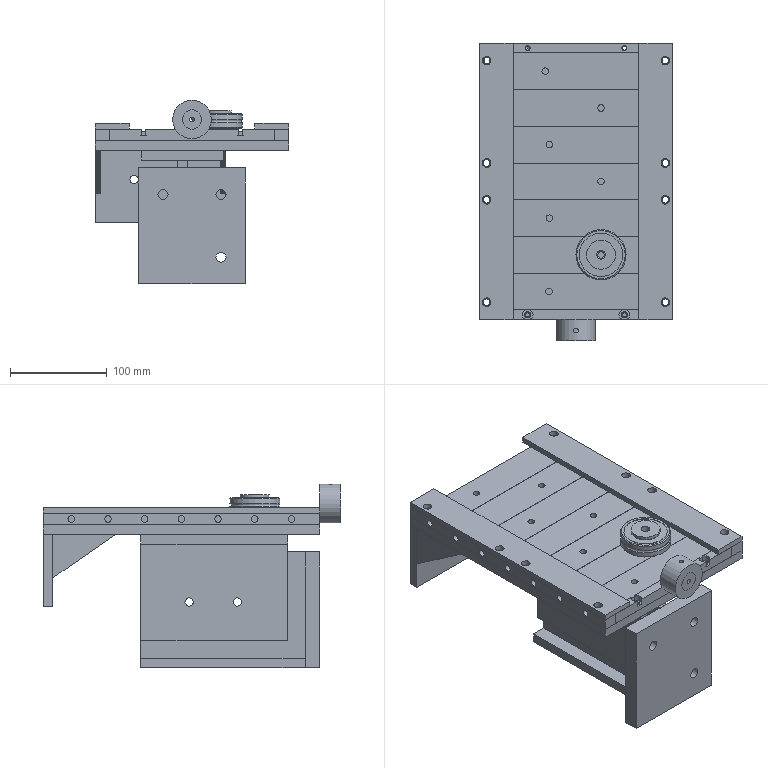Assembly | NX | mm | 25 component files | 25 solids | 279 faces | box 200 x 308 x 190.07 mm | volume 2075251 mm3 | plane 144 | cylinder 95 | cone 39 | torus 1 | commonest cylinder face diameters 6.8 x36 9 x17 10.5 x11 20 x5 4.2 x5 30 x4 11 x4 8.5 x4
Bill of materials:
unnamed part 1 | 1 |  | Long straight bar with a rectangular, nearly square cross-section. It has two sets of cross holes: one set runs through the top face and the other runs through a side face.
unnamed part 2 | 1 |  | Thick rectangular plate with two round through holes in the large face and one small hole in a long edge face.
unnamed part 3 | 1 |  | Flat rectangular plate with four round through holes, one near each corner.
unnamed part 4 | 1 |  | Thin, flat, long strip with four round through holes in a line, set off-center toward one long edge.
unnamed part 5 | 1 |  | Ring-shaped disc with a central through bore and one groove running around the outer cylindrical surface.
unnamed part 6 | 1 |  | Long rectangular bar with two vertical round holes. Each hole has a partial-depth, larger-diameter recess at the top that breaks out through one long side face, leaving a notch.
unnamed part 7 | 1 |  | Thin rectangular plate with two small round through holes, side by side, below the middle of the face.
unnamed part 8 | 1 |  | Flat right-triangle plate with a constant thickness and no holes.
unnamed part 9 | 1 |  | Thin, flat, long strip with four round through holes in a line, set off-center toward one long edge.
unnamed part 10 | 1 |  | Thick, almost square plate with three round through holes at three corners of a rectangular pattern. The fourth corner has no hole.
unnamed part 11 | 1 |  | Flat right-triangle plate with a partly open cylindrical bore running down from the top edge, near the right-angle corner.
unnamed part 12 | 1 |  | Long straight bar with a rectangular, nearly square cross-section. It has two sets of cross holes: one set runs through the top face and the other runs through a side face.
unnamed part 13 | 1 |  | Flat rectangular plate of uniform thickness with 16 round through-holes: 8 larger holes in two columns near the long edges, 4 interior holes in a rectangular pattern, and 4 smaller holes near the two short edges.
unnamed part 14 | 1 |  | Solid cylinder with a small coaxial through-bore. Its length is a little greater than its diameter, giving a thick-walled tube or spacer-like shape.
unnamed part 15 | 1 |  | Rectangular flat bar with a single round through-hole set off-center toward one end along the length, centered across the width.
unnamed part 16 | 1 |  | Flanged cylindrical bushing-like part: a thin, larger-diameter disc flange on top of a smaller-diameter cylindrical body, with a coaxial through-bore.
unnamed part 17 | 1 |  | Thin flat annular ring (washer-like): a circular disc with a large concentric through-hole.
unnamed part 18 | 6 |  | Rectangular flat bar with a single round through-hole set off-center toward one end along the length, centered across the width.
unnamed part 19 | 1 |  | L-shaped angle bracket: a tall rectangular plate with a short perpendicular foot along its bottom edge. The tall plate has two parallel elongated slots with rounded ends.
unnamed part 20 | 1 |  | Thick-walled ring or short tube with a large coaxial bore and one small radial hole through the outer wall at about mid-length (collar-like shape).
Mates:
1. fix | washer_2 1 component
2. fix | bent_shaft_2 1 component
3. fix | rolling_shaft 1 component